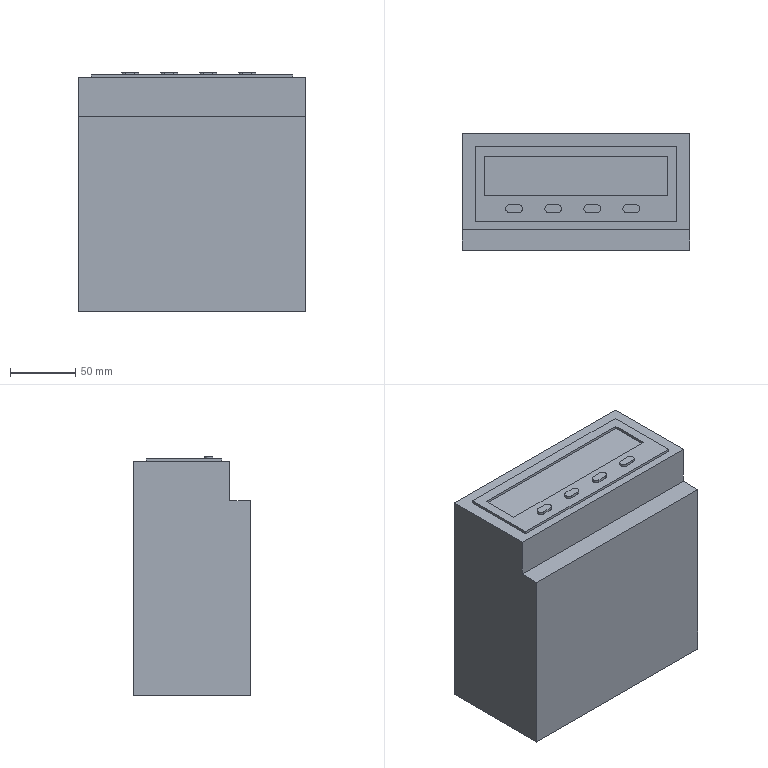Component | SolidWorks | Chassis-2 | 1 solid | 38 faces | box 175 x 90 x 184 mm | volume 2760814 mm3 | plane 30 | cylinder 8 | commonest cylinder face diameters 6 x8
build123d program:
from build123d import *

# Parameters (mm, degrees)
SKETCH1_W           = 175
SKETCH1_H           = 150
BOSS_EXTRUDE1_DEPTH = 90
SKETCH2_W           = 175
SKETCH2_H           = 73.952
BOSS_EXTRUDE2_DEPTH = 30
SKETCH3_W           = 155
SKETCH3_H           = 57.955
SKETCH3_W_2         = 141
SKETCH3_H_2         = 30
BOSS_EXTRUDE3_DEPTH = 2
BOSS_EXTRUDE4_DEPTH = 2


with BuildPart() as part:
    # Sketch1 → Boss-Extrude1 (new body)
    with BuildSketch(Plane.XY):
        with Locations((-127.5, 15)):
            Rectangle(SKETCH1_W, SKETCH1_H)
    extrude(amount=BOSS_EXTRUDE1_DEPTH)

    # Sketch2 → Boss-Extrude2 (add)
    with BuildSketch(Plane.XZ.offset(60)):
        with Locations((-127.5, 53.024)):
            Rectangle(SKETCH2_W, SKETCH2_H)
    extrude(amount=BOSS_EXTRUDE2_DEPTH)

    # Sketch3 → Boss-Extrude3 (add)
    with BuildSketch(Plane.XZ.offset(90)):
        with Locations((-127.5, 51.026)):
            Rectangle(SKETCH3_W, SKETCH3_H)
        with Locations((-127.5, 57.048)):
            Rectangle(SKETCH3_W_2, SKETCH3_H_2, mode=Mode.SUBTRACT)
    extrude(amount=BOSS_EXTRUDE3_DEPTH)

    # Sketch4 → Boss-Extrude4 (add)
    with BuildSketch(Plane.XZ.offset(92)):
        with BuildLine():
            Line((-178.5, 35.048), (-171.5, 35.048))
            ThreePointArc((-171.5, 35.048), (-168.5, 32.048), (-171.5, 29.048))
            Line((-171.5, 29.048), (-178.5, 29.048))
            ThreePointArc((-178.5, 29.048), (-181.5, 32.048), (-178.5, 35.048))
        make_face()
        with BuildLine():
            Line((-148.5, 35.048), (-141.5, 35.048))
            ThreePointArc((-141.5, 35.048), (-138.5, 32.048), (-141.5, 29.048))
            Line((-141.5, 29.048), (-148.5, 29.048))
            ThreePointArc((-148.5, 29.048), (-151.5, 32.048), (-148.5, 35.048))
        make_face()
        with BuildLine():
            Line((-118.5, 35.048), (-111.5, 35.048))
            ThreePointArc((-111.5, 35.048), (-108.5, 32.048), (-111.5, 29.048))
            Line((-111.5, 29.048), (-118.5, 29.048))
            ThreePointArc((-118.5, 29.048), (-121.5, 32.048), (-118.5, 35.048))
        make_face()
        with BuildLine():
            Line((-88.5, 35.048), (-81.5, 35.048))
            ThreePointArc((-81.5, 35.048), (-78.5, 32.048), (-81.5, 29.048))
            Line((-81.5, 29.048), (-88.5, 29.048))
            ThreePointArc((-88.5, 29.048), (-91.5, 32.048), (-88.5, 35.048))
        make_face()
    extrude(amount=BOSS_EXTRUDE4_DEPTH)


solid = part.part

# Placed as in the assembly
solid = solid.moved(Location((-695, 260, -10), (-90, 0, 0)))
STEP:
#1=COLOUR_RGB('',0.7922,0.8196,0.9333);
#2=FILL_AREA_STYLE_COLOUR('',#1);
#3=FILL_AREA_STYLE('',(#2));
#4=SURFACE_STYLE_FILL_AREA(#3);
#5=SURFACE_SIDE_STYLE('',(#4));
#6=SURFACE_STYLE_USAGE(.BOTH.,#5);
#7=PRESENTATION_STYLE_ASSIGNMENT((#6));
#8=CARTESIAN_POINT('',(-35.433,11.104,3.228));
#9=VERTEX_POINT('',#8);
#10=CARTESIAN_POINT('',(-29.331,11.104,3.228));
#11=VERTEX_POINT('',#10);
#12=CARTESIAN_POINT('',(-35.433,11.104,3.228));
#13=DIRECTION('',(1.,0.,0.));
#14=VECTOR('',#13,39.37);
#15=LINE('',#12,#14);
#16=EDGE_CURVE('',#9,#11,#15,.T.);
#17=ORIENTED_EDGE('',*,*,#16,.T.);
#18=CARTESIAN_POINT('',(-29.331,13.386,3.228));
#19=VERTEX_POINT('',#18);
#20=CARTESIAN_POINT('',(-29.331,11.104,3.228));
#21=DIRECTION('',(-0.,1.,0.));
#22=VECTOR('',#21,39.37);
#23=LINE('',#20,#22);
#24=EDGE_CURVE('',#11,#19,#23,.T.);
#25=ORIENTED_EDGE('',*,*,#24,.T.);
#26=CARTESIAN_POINT('',(-35.433,13.386,3.228));
#27=VERTEX_POINT('',#26);
#28=CARTESIAN_POINT('',(-29.331,13.386,3.228));
#29=DIRECTION('',(-1.,-0.,0.));
#30=VECTOR('',#29,39.37);
#31=LINE('',#28,#30);
#32=EDGE_CURVE('',#19,#27,#31,.T.);
#33=ORIENTED_EDGE('',*,*,#32,.T.);
#34=CARTESIAN_POINT('',(-35.433,13.386,3.228));
#35=DIRECTION('',(0.,-1.,0.));
#36=VECTOR('',#35,39.37);
#37=LINE('',#34,#36);
#38=EDGE_CURVE('',#27,#9,#37,.T.);
#39=ORIENTED_EDGE('',*,*,#38,.T.);
#40=EDGE_LOOP('',(#17,#25,#33,#39));
#41=FACE_OUTER_BOUND('',#40,.T.);
#42=CARTESIAN_POINT('',(-29.606,13.073,3.228));
#43=VERTEX_POINT('',#42);
#44=CARTESIAN_POINT('',(-35.157,13.073,3.228));
#45=VERTEX_POINT('',#44);
#46=CARTESIAN_POINT('',(-29.606,13.073,3.228));
#47=DIRECTION('',(-1.,-0.,0.));
#48=VECTOR('',#47,39.37);
#49=LINE('',#46,#48);
#50=EDGE_CURVE('',#43,#45,#49,.T.);
#51=ORIENTED_EDGE('',*,*,#50,.F.);
#52=CARTESIAN_POINT('',(-29.606,11.892,3.228));
#53=VERTEX_POINT('',#52);
#54=CARTESIAN_POINT('',(-29.606,13.073,3.228));
#55=DIRECTION('',(-0.,1.,0.));
#56=VECTOR('',#55,39.37);
#57=LINE('',#54,#56);
#58=EDGE_CURVE('',#53,#43,#57,.T.);
#59=ORIENTED_EDGE('',*,*,#58,.F.);
#60=CARTESIAN_POINT('',(-35.157,11.892,3.228));
#61=VERTEX_POINT('',#60);
#62=CARTESIAN_POINT('',(-29.606,11.892,3.228));
#63=DIRECTION('',(1.,0.,0.));
#64=VECTOR('',#63,39.37);
#65=LINE('',#62,#64);
#66=EDGE_CURVE('',#61,#53,#65,.T.);
#67=ORIENTED_EDGE('',*,*,#66,.F.);
#68=CARTESIAN_POINT('',(-35.157,13.073,3.228));
#69=DIRECTION('',(0.,-1.,0.));
#70=VECTOR('',#69,39.37);
#71=LINE('',#68,#70);
#72=EDGE_CURVE('',#45,#61,#71,.T.);
#73=ORIENTED_EDGE('',*,*,#72,.F.);
#74=EDGE_LOOP('',(#51,#59,#67,#73));
#75=FACE_BOUND('',#74,.T.);
#76=CARTESIAN_POINT('',(-34.39,11.38,3.228));
#77=VERTEX_POINT('',#76);
#78=CARTESIAN_POINT('',(-34.114,11.38,3.228));
#79=VERTEX_POINT('',#78);
#80=CARTESIAN_POINT('',(-34.39,11.38,3.228));
#81=DIRECTION('',(1.,0.,0.));
#82=VECTOR('',#81,39.37);
#83=LINE('',#80,#82);
#84=EDGE_CURVE('',#77,#79,#83,.T.);
#85=ORIENTED_EDGE('',*,*,#84,.F.);
#86=CARTESIAN_POINT('',(-34.39,11.616,3.228));
#87=VERTEX_POINT('',#86);
#88=CARTESIAN_POINT('',(-34.39,11.498,3.228));
#89=DIRECTION('',(0.,0.,1.));
#90=DIRECTION('',(0.,-1.,0.));
#91=AXIS2_PLACEMENT_3D('',#88,#89,#90);
#92=CIRCLE('',#91,0.1181);
#93=EDGE_CURVE('',#87,#77,#92,.T.);
#94=ORIENTED_EDGE('',*,*,#93,.F.);
#95=CARTESIAN_POINT('',(-34.114,11.616,3.228));
#96=VERTEX_POINT('',#95);
#97=CARTESIAN_POINT('',(-34.39,11.616,3.228));
#98=DIRECTION('',(-1.,-0.,0.));
#99=VECTOR('',#98,39.37);
#100=LINE('',#97,#99);
#101=EDGE_CURVE('',#96,#87,#100,.T.);
#102=ORIENTED_EDGE('',*,*,#101,.F.);
#103=CARTESIAN_POINT('',(-34.114,11.498,3.228));
#104=DIRECTION('',(0.,0.,1.));
#105=DIRECTION('',(0.,-1.,0.));
#106=AXIS2_PLACEMENT_3D('',#103,#104,#105);
#107=CIRCLE('',#106,0.1181);
#108=EDGE_CURVE('',#79,#96,#107,.T.);
#109=ORIENTED_EDGE('',*,*,#108,.F.);
#110=EDGE_LOOP('',(#85,#94,#102,#109));
#111=FACE_BOUND('',#110,.T.);
#112=CARTESIAN_POINT('',(-33.209,11.38,3.228));
#113=VERTEX_POINT('',#112);
#114=CARTESIAN_POINT('',(-32.933,11.38,3.228));
#115=VERTEX_POINT('',#114);
#116=CARTESIAN_POINT('',(-33.209,11.38,3.228));
#117=DIRECTION('',(1.,0.,0.));
#118=VECTOR('',#117,39.37);
#119=LINE('',#116,#118);
#120=EDGE_CURVE('',#113,#115,#119,.T.);
#121=ORIENTED_EDGE('',*,*,#120,.F.);
#122=CARTESIAN_POINT('',(-33.209,11.616,3.228));
#123=VERTEX_POINT('',#122);
#124=CARTESIAN_POINT('',(-33.209,11.498,3.228));
#125=DIRECTION('',(0.,0.,1.));
#126=DIRECTION('',(0.,-1.,0.));
#127=AXIS2_PLACEMENT_3D('',#124,#125,#126);
#128=CIRCLE('',#127,0.1181);
#129=EDGE_CURVE('',#123,#113,#128,.T.);
#130=ORIENTED_EDGE('',*,*,#129,.F.);
#131=CARTESIAN_POINT('',(-32.933,11.616,3.228));
#132=VERTEX_POINT('',#131);
#133=CARTESIAN_POINT('',(-33.209,11.616,3.228));
#134=DIRECTION('',(-1.,-0.,0.));
#135=VECTOR('',#134,39.37);
#136=LINE('',#133,#135);
#137=EDGE_CURVE('',#132,#123,#136,.T.);
#138=ORIENTED_EDGE('',*,*,#137,.F.);
#139=CARTESIAN_POINT('',(-32.933,11.498,3.228));
#140=DIRECTION('',(0.,0.,1.));
#141=DIRECTION('',(0.,-1.,0.));
#142=AXIS2_PLACEMENT_3D('',#139,#140,#141);
#143=CIRCLE('',#142,0.1181);
#144=EDGE_CURVE('',#115,#132,#143,.T.);
#145=ORIENTED_EDGE('',*,*,#144,.F.);
#146=EDGE_LOOP('',(#121,#130,#138,#145));
#147=FACE_BOUND('',#146,.T.);
#148=CARTESIAN_POINT('',(-32.028,11.38,3.228));
#149=VERTEX_POINT('',#148);
#150=CARTESIAN_POINT('',(-31.752,11.38,3.228));
#151=VERTEX_POINT('',#150);
#152=CARTESIAN_POINT('',(-32.028,11.38,3.228));
#153=DIRECTION('',(1.,0.,0.));
#154=VECTOR('',#153,39.37);
#155=LINE('',#152,#154);
#156=EDGE_CURVE('',#149,#151,#155,.T.);
#157=ORIENTED_EDGE('',*,*,#156,.F.);
#158=CARTESIAN_POINT('',(-32.028,11.616,3.228));
#159=VERTEX_POINT('',#158);
#160=CARTESIAN_POINT('',(-32.028,11.498,3.228));
#161=DIRECTION('',(0.,0.,1.));
#162=DIRECTION('',(0.,-1.,0.));
#163=AXIS2_PLACEMENT_3D('',#160,#161,#162);
#164=CIRCLE('',#163,0.1181);
#165=EDGE_CURVE('',#159,#149,#164,.T.);
#166=ORIENTED_EDGE('',*,*,#165,.F.);
#167=CARTESIAN_POINT('',(-31.752,11.616,3.228));
#168=VERTEX_POINT('',#167);
#169=CARTESIAN_POINT('',(-32.028,11.616,3.228));
#170=DIRECTION('',(-1.,-0.,0.));
#171=VECTOR('',#170,39.37);
#172=LINE('',#169,#171);
#173=EDGE_CURVE('',#168,#159,#172,.T.);
#174=ORIENTED_EDGE('',*,*,#173,.F.);
#175=CARTESIAN_POINT('',(-31.752,11.498,3.228));
#176=DIRECTION('',(0.,0.,1.));
#177=DIRECTION('',(0.,-1.,0.));
#178=AXIS2_PLACEMENT_3D('',#175,#176,#177);
#179=CIRCLE('',#178,0.1181);
#180=EDGE_CURVE('',#151,#168,#179,.T.);
#181=ORIENTED_EDGE('',*,*,#180,.F.);
#182=EDGE_LOOP('',(#157,#166,#174,#181));
#183=FACE_BOUND('',#182,.T.);
#184=CARTESIAN_POINT('',(-30.846,11.38,3.228));
#185=VERTEX_POINT('',#184);
#186=CARTESIAN_POINT('',(-30.571,11.38,3.228));
#187=VERTEX_POINT('',#186);
#188=CARTESIAN_POINT('',(-30.846,11.38,3.228));
#189=DIRECTION('',(1.,0.,0.));
#190=VECTOR('',#189,39.37);
#191=LINE('',#188,#190);
#192=EDGE_CURVE('',#185,#187,#191,.T.);
#193=ORIENTED_EDGE('',*,*,#192,.F.);
#194=CARTESIAN_POINT('',(-30.846,11.616,3.228));
#195=VERTEX_POINT('',#194);
#196=CARTESIAN_POINT('',(-30.846,11.498,3.228));
#197=DIRECTION('',(0.,0.,1.));
#198=DIRECTION('',(0.,-1.,0.));
#199=AXIS2_PLACEMENT_3D('',#196,#197,#198);
#200=CIRCLE('',#199,0.1181);
#201=EDGE_CURVE('',#195,#185,#200,.T.);
#202=ORIENTED_EDGE('',*,*,#201,.F.);
#203=CARTESIAN_POINT('',(-30.571,11.616,3.228));
#204=VERTEX_POINT('',#203);
#205=CARTESIAN_POINT('',(-30.846,11.616,3.228));
#206=DIRECTION('',(-1.,-0.,0.));
#207=VECTOR('',#206,39.37);
#208=LINE('',#205,#207);
#209=EDGE_CURVE('',#204,#195,#208,.T.);
#210=ORIENTED_EDGE('',*,*,#209,.F.);
#211=CARTESIAN_POINT('',(-30.571,11.498,3.228));
#212=DIRECTION('',(0.,0.,1.));
#213=DIRECTION('',(0.,-1.,0.));
#214=AXIS2_PLACEMENT_3D('',#211,#212,#213);
#215=CIRCLE('',#214,0.1181);
#216=EDGE_CURVE('',#187,#204,#215,.T.);
#217=ORIENTED_EDGE('',*,*,#216,.F.);
#218=EDGE_LOOP('',(#193,#202,#210,#217));
#219=FACE_BOUND('',#218,.T.);
#220=CARTESIAN_POINT('',(-27.362,10.236,3.228));
#221=DIRECTION('',(0.,0.,1.));
#222=DIRECTION('',(0.,-1.,0.));
#223=AXIS2_PLACEMENT_3D('',#220,#221,#222);
#224=PLANE('',#223);
#225=ADVANCED_FACE('',(#41,#75,#111,#147,#183,#219),#224,.T.);
#226=CARTESIAN_POINT('',(-28.937,10.868,3.15));
#227=VERTEX_POINT('',#226);
#228=CARTESIAN_POINT('',(-28.937,13.78,3.15));
#229=VERTEX_POINT('',#228);
#230=CARTESIAN_POINT('',(-28.937,13.78,3.15));
#231=DIRECTION('',(-0.,1.,0.));
#232=VECTOR('',#231,39.37);
#233=LINE('',#230,#232);
#234=EDGE_CURVE('',#227,#229,#233,.T.);
#235=ORIENTED_EDGE('',*,*,#234,.T.);
#236=CARTESIAN_POINT('',(-35.827,13.78,3.15));
#237=VERTEX_POINT('',#236);
#238=CARTESIAN_POINT('',(-28.937,13.78,3.15));
#239=DIRECTION('',(-1.,-0.,0.));
#240=VECTOR('',#239,39.37);
#241=LINE('',#238,#240);
#242=EDGE_CURVE('',#229,#237,#241,.T.);
#243=ORIENTED_EDGE('',*,*,#242,.T.);
#244=CARTESIAN_POINT('',(-35.827,10.868,3.15));
#245=VERTEX_POINT('',#244);
#246=CARTESIAN_POINT('',(-35.827,13.78,3.15));
#247=DIRECTION('',(-0.,-1.,0.));
#248=VECTOR('',#247,39.37);
#249=LINE('',#246,#248);
#250=EDGE_CURVE('',#237,#245,#249,.T.);
#251=ORIENTED_EDGE('',*,*,#250,.T.);
#252=CARTESIAN_POINT('',(-28.937,10.868,3.15));
#253=DIRECTION('',(1.,0.,0.));
#254=VECTOR('',#253,39.37);
#255=LINE('',#252,#254);
#256=EDGE_CURVE('',#245,#227,#255,.T.);
#257=ORIENTED_EDGE('',*,*,#256,.T.);
#258=EDGE_LOOP('',(#235,#243,#251,#257));
#259=FACE_OUTER_BOUND('',#258,.T.);
#260=CARTESIAN_POINT('',(-35.433,11.104,3.15));
#261=VERTEX_POINT('',#260);
#262=CARTESIAN_POINT('',(-29.331,11.104,3.15));
#263=VERTEX_POINT('',#262);
#264=CARTESIAN_POINT('',(-35.433,11.104,3.15));
#265=DIRECTION('',(1.,0.,0.));
#266=VECTOR('',#265,39.37);
#267=LINE('',#264,#266);
#268=EDGE_CURVE('',#261,#263,#267,.T.);
#269=ORIENTED_EDGE('',*,*,#268,.F.);
#270=CARTESIAN_POINT('',(-35.433,13.386,3.15));
#271=VERTEX_POINT('',#270);
#272=CARTESIAN_POINT('',(-35.433,13.386,3.15));
#273=DIRECTION('',(0.,-1.,0.));
#274=VECTOR('',#273,39.37);
#275=LINE('',#272,#274);
#276=EDGE_CURVE('',#271,#261,#275,.T.);
#277=ORIENTED_EDGE('',*,*,#276,.F.);
#278=CARTESIAN_POINT('',(-29.331,13.386,3.15));
#279=VERTEX_POINT('',#278);
#280=CARTESIAN_POINT('',(-29.331,13.386,3.15));
#281=DIRECTION('',(-1.,-0.,0.));
#282=VECTOR('',#281,39.37);
#283=LINE('',#280,#282);
#284=EDGE_CURVE('',#279,#271,#283,.T.);
#285=ORIENTED_EDGE('',*,*,#284,.F.);
#286=CARTESIAN_POINT('',(-29.331,11.104,3.15));
#287=DIRECTION('',(-0.,1.,0.));
#288=VECTOR('',#287,39.37);
#289=LINE('',#286,#288);
#290=EDGE_CURVE('',#263,#279,#289,.T.);
#291=ORIENTED_EDGE('',*,*,#290,.F.);
#292=EDGE_LOOP('',(#269,#277,#285,#291));
#293=FACE_BOUND('',#292,.T.);
#294=CARTESIAN_POINT('',(-27.362,10.236,3.15));
#295=DIRECTION('',(0.,0.,-1.));
#296=DIRECTION('',(-0.,1.,0.));
#297=AXIS2_PLACEMENT_3D('',#294,#295,#296);
#298=PLANE('',#297);
#299=ADVANCED_FACE('',(#259,#293),#298,.F.);
#300=CARTESIAN_POINT('',(-35.827,10.868,1.969));
#301=VERTEX_POINT('',#300);
#302=CARTESIAN_POINT('',(-28.937,10.868,1.969));
#303=VERTEX_POINT('',#302);
#304=CARTESIAN_POINT('',(-28.937,10.868,1.969));
#305=DIRECTION('',(1.,0.,0.));
#306=VECTOR('',#305,39.37);
#307=LINE('',#304,#306);
#308=EDGE_CURVE('',#301,#303,#307,.T.);
#309=ORIENTED_EDGE('',*,*,#308,.F.);
#310=CARTESIAN_POINT('',(-35.827,10.236,1.969));
#311=VERTEX_POINT('',#310);
#312=CARTESIAN_POINT('',(-35.827,13.78,1.969));
#313=DIRECTION('',(0.,-1.,0.));
#314=VECTOR('',#313,39.37);
#315=LINE('',#312,#314);
#316=EDGE_CURVE('',#301,#311,#315,.T.);
#317=ORIENTED_EDGE('',*,*,#316,.T.);
#318=CARTESIAN_POINT('',(-28.937,10.236,1.969));
#319=VERTEX_POINT('',#318);
#320=CARTESIAN_POINT('',(-35.827,10.236,1.969));
#321=DIRECTION('',(1.,0.,-0.));
#322=VECTOR('',#321,39.37);
#323=LINE('',#320,#322);
#324=EDGE_CURVE('',#311,#319,#323,.T.);
#325=ORIENTED_EDGE('',*,*,#324,.T.);
#326=CARTESIAN_POINT('',(-28.937,13.78,1.969));
#327=DIRECTION('',(0.,-1.,0.));
#328=VECTOR('',#327,39.37);
#329=LINE('',#326,#328);
#330=EDGE_CURVE('',#303,#319,#329,.T.);
#331=ORIENTED_EDGE('',*,*,#330,.F.);
#332=EDGE_LOOP('',(#309,#317,#325,#331));
#333=FACE_OUTER_BOUND('',#332,.T.);
#334=CARTESIAN_POINT('',(-35.827,13.78,1.969));
#335=DIRECTION('',(-0.,-0.,-1.));
#336=DIRECTION('',(-1.,-0.,0.));
#337=AXIS2_PLACEMENT_3D('',#334,#335,#336);
#338=PLANE('',#337);
#339=ADVANCED_FACE('',(#333),#338,.F.);
#340=CARTESIAN_POINT('',(-35.827,10.236,-3.937));
#341=VERTEX_POINT('',#340);
#342=CARTESIAN_POINT('',(-35.827,10.236,-3.937));
#343=DIRECTION('',(0.,0.,1.));
#344=VECTOR('',#343,39.37);
#345=LINE('',#342,#344);
#346=EDGE_CURVE('',#341,#311,#345,.T.);
#347=ORIENTED_EDGE('',*,*,#346,.T.);
#348=ORIENTED_EDGE('',*,*,#316,.F.);
#349=CARTESIAN_POINT('',(-35.827,10.868,3.15));
#350=DIRECTION('',(0.,0.,-1.));
#351=VECTOR('',#350,39.37);
#352=LINE('',#349,#351);
#353=EDGE_CURVE('',#245,#301,#352,.T.);
#354=ORIENTED_EDGE('',*,*,#353,.F.);
#355=ORIENTED_EDGE('',*,*,#250,.F.);
#356=CARTESIAN_POINT('',(-35.827,13.78,-3.937));
#357=VERTEX_POINT('',#356);
#358=CARTESIAN_POINT('',(-35.827,13.78,-3.937));
#359=DIRECTION('',(0.,0.,1.));
#360=VECTOR('',#359,39.37);
#361=LINE('',#358,#360);
#362=EDGE_CURVE('',#357,#237,#361,.T.);
#363=ORIENTED_EDGE('',*,*,#362,.F.);
#364=CARTESIAN_POINT('',(-35.827,13.78,-3.937));
#365=DIRECTION('',(0.,-1.,0.));
#366=VECTOR('',#365,39.37);
#367=LINE('',#364,#366);
#368=EDGE_CURVE('',#357,#341,#367,.T.);
#369=ORIENTED_EDGE('',*,*,#368,.T.);
#370=EDGE_LOOP('',(#347,#348,#354,#355,#363,#369));
#371=FACE_OUTER_BOUND('',#370,.T.);
#372=CARTESIAN_POINT('',(-35.827,13.78,-3.937));
#373=DIRECTION('',(1.,0.,-0.));
#374=DIRECTION('',(-0.,-0.,-1.));
#375=AXIS2_PLACEMENT_3D('',#372,#373,#374);
#376=PLANE('',#375);
#377=ADVANCED_FACE('',(#371),#376,.F.);
#378=CARTESIAN_POINT('',(-28.937,10.236,-3.937));
#379=VERTEX_POINT('',#378);
#380=CARTESIAN_POINT('',(-28.937,10.236,-3.937));
#381=DIRECTION('',(-0.,-0.,-1.));
#382=VECTOR('',#381,39.37);
#383=LINE('',#380,#382);
#384=EDGE_CURVE('',#319,#379,#383,.T.);
#385=ORIENTED_EDGE('',*,*,#384,.T.);
#386=CARTESIAN_POINT('',(-28.937,13.78,-3.937));
#387=VERTEX_POINT('',#386);
#388=CARTESIAN_POINT('',(-28.937,13.78,-3.937));
#389=DIRECTION('',(0.,-1.,0.));
#390=VECTOR('',#389,39.37);
#391=LINE('',#388,#390);
#392=EDGE_CURVE('',#387,#379,#391,.T.);
#393=ORIENTED_EDGE('',*,*,#392,.F.);
#394=CARTESIAN_POINT('',(-28.937,13.78,-3.937));
#395=DIRECTION('',(-0.,-0.,-1.));
#396=VECTOR('',#395,39.37);
#397=LINE('',#394,#396);
#398=EDGE_CURVE('',#229,#387,#397,.T.);
#399=ORIENTED_EDGE('',*,*,#398,.F.);
#400=ORIENTED_EDGE('',*,*,#234,.F.);
#401=CARTESIAN_POINT('',(-28.937,10.868,3.15));
#402=DIRECTION('',(0.,0.,-1.));
#403=VECTOR('',#402,39.37);
#404=LINE('',#401,#403);
#405=EDGE_CURVE('',#227,#303,#404,.T.);
#406=ORIENTED_EDGE('',*,*,#405,.T.);
#407=ORIENTED_EDGE('',*,*,#330,.T.);
#408=EDGE_LOOP('',(#385,#393,#399,#400,#406,#407));
#409=FACE_OUTER_BOUND('',#408,.T.);
#410=CARTESIAN_POINT('',(-28.937,13.78,-3.937));
#411=DIRECTION('',(-1.,-0.,0.));
#412=DIRECTION('',(0.,0.,1.));
#413=AXIS2_PLACEMENT_3D('',#410,#411,#412);
#414=PLANE('',#413);
#415=ADVANCED_FACE('',(#409),#414,.F.);
#416=CARTESIAN_POINT('',(-35.827,10.236,-3.937));
#417=DIRECTION('',(-1.,-0.,0.));
#418=VECTOR('',#417,39.37);
#419=LINE('',#416,#418);
#420=EDGE_CURVE('',#379,#341,#419,.T.);
#421=ORIENTED_EDGE('',*,*,#420,.T.);
#422=ORIENTED_EDGE('',*,*,#368,.F.);
#423=CARTESIAN_POINT('',(-35.827,13.78,-3.937));
#424=DIRECTION('',(-1.,-0.,0.));
#425=VECTOR('',#424,39.37);
#426=LINE('',#423,#425);
#427=EDGE_CURVE('',#387,#357,#426,.T.);
#428=ORIENTED_EDGE('',*,*,#427,.F.);
#429=ORIENTED_EDGE('',*,*,#392,.T.);
#430=EDGE_LOOP('',(#421,#422,#428,#429));
#431=FACE_OUTER_BOUND('',#430,.T.);
#432=CARTESIAN_POINT('',(-35.827,13.78,-3.937));
#433=DIRECTION('',(0.,0.,1.));
#434=DIRECTION('',(0.,-1.,0.));
#435=AXIS2_PLACEMENT_3D('',#432,#433,#434);
#436=PLANE('',#435);
#437=ADVANCED_FACE('',(#431),#436,.F.);
#438=ORIENTED_EDGE('',*,*,#362,.T.);
#439=ORIENTED_EDGE('',*,*,#242,.F.);
#440=ORIENTED_EDGE('',*,*,#398,.T.);
#441=ORIENTED_EDGE('',*,*,#427,.T.);
#442=EDGE_LOOP('',(#438,#439,#440,#441));
#443=FACE_OUTER_BOUND('',#442,.T.);
#444=CARTESIAN_POINT('',(-27.362,13.78,-0.3937));
#445=DIRECTION('',(-0.,1.,0.));
#446=DIRECTION('',(1.,0.,0.));
#447=AXIS2_PLACEMENT_3D('',#444,#445,#446);
#448=PLANE('',#447);
#449=ADVANCED_FACE('',(#443),#448,.T.);
#450=ORIENTED_EDGE('',*,*,#346,.F.);
#451=ORIENTED_EDGE('',*,*,#420,.F.);
#452=ORIENTED_EDGE('',*,*,#384,.F.);
#453=ORIENTED_EDGE('',*,*,#324,.F.);
#454=EDGE_LOOP('',(#450,#451,#452,#453));
#455=FACE_OUTER_BOUND('',#454,.T.);
#456=CARTESIAN_POINT('',(-27.362,10.236,-0.3937));
#457=DIRECTION('',(-0.,1.,0.));
#458=DIRECTION('',(1.,0.,0.));
#459=AXIS2_PLACEMENT_3D('',#456,#457,#458);
#460=PLANE('',#459);
#461=ADVANCED_FACE('',(#455),#460,.F.);
#462=ORIENTED_EDGE('',*,*,#308,.T.);
#463=ORIENTED_EDGE('',*,*,#405,.F.);
#464=ORIENTED_EDGE('',*,*,#256,.F.);
#465=ORIENTED_EDGE('',*,*,#353,.T.);
#466=EDGE_LOOP('',(#462,#463,#464,#465));
#467=FACE_OUTER_BOUND('',#466,.T.);
#468=CARTESIAN_POINT('',(-28.937,10.868,3.15));
#469=DIRECTION('',(-0.,1.,0.));
#470=DIRECTION('',(1.,0.,0.));
#471=AXIS2_PLACEMENT_3D('',#468,#469,#470);
#472=PLANE('',#471);
#473=ADVANCED_FACE('',(#467),#472,.F.);
#474=ORIENTED_EDGE('',*,*,#268,.T.);
#475=CARTESIAN_POINT('',(-29.331,11.104,3.228));
#476=DIRECTION('',(0.,0.,-1.));
#477=VECTOR('',#476,39.37);
#478=LINE('',#475,#477);
#479=EDGE_CURVE('',#11,#263,#478,.T.);
#480=ORIENTED_EDGE('',*,*,#479,.F.);
#481=ORIENTED_EDGE('',*,*,#16,.F.);
#482=CARTESIAN_POINT('',(-35.433,11.104,3.228));
#483=DIRECTION('',(0.,0.,-1.));
#484=VECTOR('',#483,39.37);
#485=LINE('',#482,#484);
#486=EDGE_CURVE('',#9,#261,#485,.T.);
#487=ORIENTED_EDGE('',*,*,#486,.T.);
#488=EDGE_LOOP('',(#474,#480,#481,#487));
#489=FACE_OUTER_BOUND('',#488,.T.);
#490=CARTESIAN_POINT('',(-35.433,11.104,3.228));
#491=DIRECTION('',(-0.,1.,0.));
#492=DIRECTION('',(1.,0.,0.));
#493=AXIS2_PLACEMENT_3D('',#490,#491,#492);
#494=PLANE('',#493);
#495=ADVANCED_FACE('',(#489),#494,.F.);
#496=ORIENTED_EDGE('',*,*,#290,.T.);
#497=CARTESIAN_POINT('',(-29.331,13.386,3.228));
#498=DIRECTION('',(0.,0.,-1.));
#499=VECTOR('',#498,39.37);
#500=LINE('',#497,#499);
#501=EDGE_CURVE('',#19,#279,#500,.T.);
#502=ORIENTED_EDGE('',*,*,#501,.F.);
#503=ORIENTED_EDGE('',*,*,#24,.F.);
#504=ORIENTED_EDGE('',*,*,#479,.T.);
#505=EDGE_LOOP('',(#496,#502,#503,#504));
#506=FACE_OUTER_BOUND('',#505,.T.);
#507=CARTESIAN_POINT('',(-29.331,11.104,3.228));
#508=DIRECTION('',(-1.,-0.,0.));
#509=DIRECTION('',(-0.,1.,0.));
#510=AXIS2_PLACEMENT_3D('',#507,#508,#509);
#511=PLANE('',#510);
#512=ADVANCED_FACE('',(#506),#511,.F.);
#513=ORIENTED_EDGE('',*,*,#284,.T.);
#514=CARTESIAN_POINT('',(-35.433,13.386,3.228));
#515=DIRECTION('',(0.,0.,-1.));
#516=VECTOR('',#515,39.37);
#517=LINE('',#514,#516);
#518=EDGE_CURVE('',#27,#271,#517,.T.);
#519=ORIENTED_EDGE('',*,*,#518,.F.);
#520=ORIENTED_EDGE('',*,*,#32,.F.);
#521=ORIENTED_EDGE('',*,*,#501,.T.);
#522=EDGE_LOOP('',(#513,#519,#520,#521));
#523=FACE_OUTER_BOUND('',#522,.T.);
#524=CARTESIAN_POINT('',(-29.331,13.386,3.228));
#525=DIRECTION('',(0.,-1.,0.));
#526=DIRECTION('',(-1.,-0.,0.));
#527=AXIS2_PLACEMENT_3D('',#524,#525,#526);
#528=PLANE('',#527);
#529=ADVANCED_FACE('',(#523),#528,.F.);
#530=ORIENTED_EDGE('',*,*,#276,.T.);
#531=ORIENTED_EDGE('',*,*,#486,.F.);
#532=ORIENTED_EDGE('',*,*,#38,.F.);
#533=ORIENTED_EDGE('',*,*,#518,.T.);
#534=EDGE_LOOP('',(#530,#531,#532,#533));
#535=FACE_OUTER_BOUND('',#534,.T.);
#536=CARTESIAN_POINT('',(-35.433,13.386,3.228));
#537=DIRECTION('',(1.,0.,0.));
#538=DIRECTION('',(0.,-1.,0.));
#539=AXIS2_PLACEMENT_3D('',#536,#537,#538);
#540=PLANE('',#539);
#541=ADVANCED_FACE('',(#535),#540,.F.);
#542=CARTESIAN_POINT('',(-29.606,11.892,3.15));
#543=VERTEX_POINT('',#542);
#544=CARTESIAN_POINT('',(-29.606,13.073,3.15));
#545=VERTEX_POINT('',#544);
#546=CARTESIAN_POINT('',(-29.606,13.073,3.15));
#547=DIRECTION('',(-0.,1.,0.));
#548=VECTOR('',#547,39.37);
#549=LINE('',#546,#548);
#550=EDGE_CURVE('',#543,#545,#549,.T.);
#551=ORIENTED_EDGE('',*,*,#550,.F.);
#552=CARTESIAN_POINT('',(-29.606,11.892,3.228));
#553=DIRECTION('',(0.,0.,-1.));
#554=VECTOR('',#553,39.37);
#555=LINE('',#552,#554);
#556=EDGE_CURVE('',#53,#543,#555,.T.);
#557=ORIENTED_EDGE('',*,*,#556,.F.);
#558=ORIENTED_EDGE('',*,*,#58,.T.);
#559=CARTESIAN_POINT('',(-29.606,13.073,3.228));
#560=DIRECTION('',(0.,0.,-1.));
#561=VECTOR('',#560,39.37);
#562=LINE('',#559,#561);
#563=EDGE_CURVE('',#43,#545,#562,.T.);
#564=ORIENTED_EDGE('',*,*,#563,.T.);
#565=EDGE_LOOP('',(#551,#557,#558,#564));
#566=FACE_OUTER_BOUND('',#565,.T.);
#567=CARTESIAN_POINT('',(-29.606,13.073,3.228));
#568=DIRECTION('',(-1.,-0.,0.));
#569=DIRECTION('',(-0.,1.,0.));
#570=AXIS2_PLACEMENT_3D('',#567,#568,#569);
#571=PLANE('',#570);
#572=ADVANCED_FACE('',(#566),#571,.T.);
#573=CARTESIAN_POINT('',(-35.157,13.073,3.15));
#574=VERTEX_POINT('',#573);
#575=CARTESIAN_POINT('',(-29.606,13.073,3.15));
#576=DIRECTION('',(-1.,-0.,0.));
#577=VECTOR('',#576,39.37);
#578=LINE('',#575,#577);
#579=EDGE_CURVE('',#545,#574,#578,.T.);
#580=ORIENTED_EDGE('',*,*,#579,.F.);
#581=ORIENTED_EDGE('',*,*,#563,.F.);
#582=ORIENTED_EDGE('',*,*,#50,.T.);
#583=CARTESIAN_POINT('',(-35.157,13.073,3.228));
#584=DIRECTION('',(0.,0.,-1.));
#585=VECTOR('',#584,39.37);
#586=LINE('',#583,#585);
#587=EDGE_CURVE('',#45,#574,#586,.T.);
#588=ORIENTED_EDGE('',*,*,#587,.T.);
#589=EDGE_LOOP('',(#580,#581,#582,#588));
#590=FACE_OUTER_BOUND('',#589,.T.);
#591=CARTESIAN_POINT('',(-29.606,13.073,3.228));
#592=DIRECTION('',(0.,-1.,0.));
#593=DIRECTION('',(-1.,-0.,0.));
#594=AXIS2_PLACEMENT_3D('',#591,#592,#593);
#595=PLANE('',#594);
#596=ADVANCED_FACE('',(#590),#595,.T.);
#597=CARTESIAN_POINT('',(-35.157,11.892,3.15));
#598=VERTEX_POINT('',#597);
#599=CARTESIAN_POINT('',(-35.157,13.073,3.15));
#600=DIRECTION('',(0.,-1.,0.));
#601=VECTOR('',#600,39.37);
#602=LINE('',#599,#601);
#603=EDGE_CURVE('',#574,#598,#602,.T.);
#604=ORIENTED_EDGE('',*,*,#603,.F.);
#605=ORIENTED_EDGE('',*,*,#587,.F.);
#606=ORIENTED_EDGE('',*,*,#72,.T.);
#607=CARTESIAN_POINT('',(-35.157,11.892,3.228));
#608=DIRECTION('',(0.,0.,-1.));
#609=VECTOR('',#608,39.37);
#610=LINE('',#607,#609);
#611=EDGE_CURVE('',#61,#598,#610,.T.);
#612=ORIENTED_EDGE('',*,*,#611,.T.);
#613=EDGE_LOOP('',(#604,#605,#606,#612));
#614=FACE_OUTER_BOUND('',#613,.T.);
#615=CARTESIAN_POINT('',(-35.157,13.073,3.228));
#616=DIRECTION('',(1.,0.,0.));
#617=DIRECTION('',(0.,-1.,0.));
#618=AXIS2_PLACEMENT_3D('',#615,#616,#617);
#619=PLANE('',#618);
#620=ADVANCED_FACE('',(#614),#619,.T.);
#621=CARTESIAN_POINT('',(-29.606,11.892,3.15));
#622=DIRECTION('',(1.,0.,0.));
#623=VECTOR('',#622,39.37);
#624=LINE('',#621,#623);
#625=EDGE_CURVE('',#598,#543,#624,.T.);
#626=ORIENTED_EDGE('',*,*,#625,.F.);
#627=ORIENTED_EDGE('',*,*,#611,.F.);
#628=ORIENTED_EDGE('',*,*,#66,.T.);
#629=ORIENTED_EDGE('',*,*,#556,.T.);
#630=EDGE_LOOP('',(#626,#627,#628,#629));
#631=FACE_OUTER_BOUND('',#630,.T.);
#632=CARTESIAN_POINT('',(-29.606,11.892,3.228));
#633=DIRECTION('',(-0.,1.,0.));
#634=DIRECTION('',(1.,0.,0.));
#635=AXIS2_PLACEMENT_3D('',#632,#633,#634);
#636=PLANE('',#635);
#637=ADVANCED_FACE('',(#631),#636,.T.);
#638=ORIENTED_EDGE('',*,*,#625,.T.);
#639=ORIENTED_EDGE('',*,*,#550,.T.);
#640=ORIENTED_EDGE('',*,*,#579,.T.);
#641=ORIENTED_EDGE('',*,*,#603,.T.);
#642=EDGE_LOOP('',(#638,#639,#640,#641));
#643=FACE_OUTER_BOUND('',#642,.T.);
#644=CARTESIAN_POINT('',(-27.362,10.236,3.15));
#645=DIRECTION('',(0.,0.,-1.));
#646=DIRECTION('',(-0.,1.,0.));
#647=AXIS2_PLACEMENT_3D('',#644,#645,#646);
#648=PLANE('',#647);
#649=ADVANCED_FACE('',(#643),#648,.F.);
#650=ORIENTED_EDGE('',*,*,#93,.T.);
#651=CARTESIAN_POINT('',(-34.39,11.38,3.307));
#652=VERTEX_POINT('',#651);
#653=CARTESIAN_POINT('',(-34.39,11.38,3.307));
#654=DIRECTION('',(0.,0.,-1.));
#655=VECTOR('',#654,39.37);
#656=LINE('',#653,#655);
#657=EDGE_CURVE('',#652,#77,#656,.T.);
#658=ORIENTED_EDGE('',*,*,#657,.F.);
#659=CARTESIAN_POINT('',(-34.39,11.616,3.307));
#660=VERTEX_POINT('',#659);
#661=CARTESIAN_POINT('',(-34.39,11.498,3.307));
#662=DIRECTION('',(0.,0.,1.));
#663=DIRECTION('',(0.,-1.,0.));
#664=AXIS2_PLACEMENT_3D('',#661,#662,#663);
#665=CIRCLE('',#664,0.1181);
#666=EDGE_CURVE('',#660,#652,#665,.T.);
#667=ORIENTED_EDGE('',*,*,#666,.F.);
#668=CARTESIAN_POINT('',(-34.39,11.616,3.307));
#669=DIRECTION('',(0.,0.,-1.));
#670=VECTOR('',#669,39.37);
#671=LINE('',#668,#670);
#672=EDGE_CURVE('',#660,#87,#671,.T.);
#673=ORIENTED_EDGE('',*,*,#672,.T.);
#674=EDGE_LOOP('',(#650,#658,#667,#673));
#675=FACE_OUTER_BOUND('',#674,.T.);
#676=CARTESIAN_POINT('',(-34.39,11.498,3.307));
#677=DIRECTION('',(0.,0.,-1.));
#678=DIRECTION('',(0.,1.,0.));
#679=AXIS2_PLACEMENT_3D('',#676,#677,#678);
#680=CYLINDRICAL_SURFACE('',#679,0.1181);
#681=ADVANCED_FACE('',(#675),#680,.T.);
#682=ORIENTED_EDGE('',*,*,#84,.T.);
#683=CARTESIAN_POINT('',(-34.114,11.38,3.307));
#684=VERTEX_POINT('',#683);
#685=CARTESIAN_POINT('',(-34.114,11.38,3.307));
#686=DIRECTION('',(0.,0.,-1.));
#687=VECTOR('',#686,39.37);
#688=LINE('',#685,#687);
#689=EDGE_CURVE('',#684,#79,#688,.T.);
#690=ORIENTED_EDGE('',*,*,#689,.F.);
#691=CARTESIAN_POINT('',(-34.39,11.38,3.307));
#692=DIRECTION('',(1.,0.,0.));
#693=VECTOR('',#692,39.37);
#694=LINE('',#691,#693);
#695=EDGE_CURVE('',#652,#684,#694,.T.);
#696=ORIENTED_EDGE('',*,*,#695,.F.);
#697=ORIENTED_EDGE('',*,*,#657,.T.);
#698=EDGE_LOOP('',(#682,#690,#696,#697));
#699=FACE_OUTER_BOUND('',#698,.T.);
#700=CARTESIAN_POINT('',(-34.39,11.38,3.307));
#701=DIRECTION('',(-0.,1.,0.));
#702=DIRECTION('',(1.,0.,0.));
#703=AXIS2_PLACEMENT_3D('',#700,#701,#702);
#704=PLANE('',#703);
#705=ADVANCED_FACE('',(#699),#704,.F.);
#706=ORIENTED_EDGE('',*,*,#108,.T.);
#707=CARTESIAN_POINT('',(-34.114,11.616,3.307));
#708=VERTEX_POINT('',#707);
#709=CARTESIAN_POINT('',(-34.114,11.616,3.307));
#710=DIRECTION('',(0.,0.,-1.));
#711=VECTOR('',#710,39.37);
#712=LINE('',#709,#711);
#713=EDGE_CURVE('',#708,#96,#712,.T.);
#714=ORIENTED_EDGE('',*,*,#713,.F.);
#715=CARTESIAN_POINT('',(-34.114,11.498,3.307));
#716=DIRECTION('',(0.,0.,1.));
#717=DIRECTION('',(0.,-1.,0.));
#718=AXIS2_PLACEMENT_3D('',#715,#716,#717);
#719=CIRCLE('',#718,0.1181);
#720=EDGE_CURVE('',#684,#708,#719,.T.);
#721=ORIENTED_EDGE('',*,*,#720,.F.);
#722=ORIENTED_EDGE('',*,*,#689,.T.);
#723=EDGE_LOOP('',(#706,#714,#721,#722));
#724=FACE_OUTER_BOUND('',#723,.T.);
#725=CARTESIAN_POINT('',(-34.114,11.498,3.307));
#726=DIRECTION('',(0.,0.,-1.));
#727=DIRECTION('',(0.,1.,0.));
#728=AXIS2_PLACEMENT_3D('',#725,#726,#727);
#729=CYLINDRICAL_SURFACE('',#728,0.1181);
#730=ADVANCED_FACE('',(#724),#729,.T.);
#731=ORIENTED_EDGE('',*,*,#101,.T.);
#732=ORIENTED_EDGE('',*,*,#672,.F.);
#733=CARTESIAN_POINT('',(-34.39,11.616,3.307));
#734=DIRECTION('',(-1.,-0.,0.));
#735=VECTOR('',#734,39.37);
#736=LINE('',#733,#735);
#737=EDGE_CURVE('',#708,#660,#736,.T.);
#738=ORIENTED_EDGE('',*,*,#737,.F.);
#739=ORIENTED_EDGE('',*,*,#713,.T.);
#740=EDGE_LOOP('',(#731,#732,#738,#739));
#741=FACE_OUTER_BOUND('',#740,.T.);
#742=CARTESIAN_POINT('',(-34.39,11.616,3.307));
#743=DIRECTION('',(0.,-1.,0.));
#744=DIRECTION('',(-1.,-0.,0.));
#745=AXIS2_PLACEMENT_3D('',#742,#743,#744);
#746=PLANE('',#745);
#747=ADVANCED_FACE('',(#741),#746,.F.);
#748=ORIENTED_EDGE('',*,*,#666,.T.);
#749=ORIENTED_EDGE('',*,*,#695,.T.);
#750=ORIENTED_EDGE('',*,*,#720,.T.);
#751=ORIENTED_EDGE('',*,*,#737,.T.);
#752=EDGE_LOOP('',(#748,#749,#750,#751));
#753=FACE_OUTER_BOUND('',#752,.T.);
#754=CARTESIAN_POINT('',(-34.39,11.498,3.307));
#755=DIRECTION('',(0.,0.,1.));
#756=DIRECTION('',(0.,-1.,0.));
#757=AXIS2_PLACEMENT_3D('',#754,#755,#756);
#758=PLANE('',#757);
#759=ADVANCED_FACE('',(#753),#758,.T.);
#760=ORIENTED_EDGE('',*,*,#129,.T.);
#761=CARTESIAN_POINT('',(-33.209,11.38,3.307));
#762=VERTEX_POINT('',#761);
#763=CARTESIAN_POINT('',(-33.209,11.38,3.307));
#764=DIRECTION('',(0.,0.,-1.));
#765=VECTOR('',#764,39.37);
#766=LINE('',#763,#765);
#767=EDGE_CURVE('',#762,#113,#766,.T.);
#768=ORIENTED_EDGE('',*,*,#767,.F.);
#769=CARTESIAN_POINT('',(-33.209,11.616,3.307));
#770=VERTEX_POINT('',#769);
#771=CARTESIAN_POINT('',(-33.209,11.498,3.307));
#772=DIRECTION('',(0.,0.,1.));
#773=DIRECTION('',(0.,-1.,0.));
#774=AXIS2_PLACEMENT_3D('',#771,#772,#773);
#775=CIRCLE('',#774,0.1181);
#776=EDGE_CURVE('',#770,#762,#775,.T.);
#777=ORIENTED_EDGE('',*,*,#776,.F.);
#778=CARTESIAN_POINT('',(-33.209,11.616,3.307));
#779=DIRECTION('',(0.,0.,-1.));
#780=VECTOR('',#779,39.37);
#781=LINE('',#778,#780);
#782=EDGE_CURVE('',#770,#123,#781,.T.);
#783=ORIENTED_EDGE('',*,*,#782,.T.);
#784=EDGE_LOOP('',(#760,#768,#777,#783));
#785=FACE_OUTER_BOUND('',#784,.T.);
#786=CARTESIAN_POINT('',(-33.209,11.498,3.307));
#787=DIRECTION('',(0.,0.,-1.));
#788=DIRECTION('',(0.,1.,0.));
#789=AXIS2_PLACEMENT_3D('',#786,#787,#788);
#790=CYLINDRICAL_SURFACE('',#789,0.1181);
#791=ADVANCED_FACE('',(#785),#790,.T.);
#792=ORIENTED_EDGE('',*,*,#120,.T.);
#793=CARTESIAN_POINT('',(-32.933,11.38,3.307));
#794=VERTEX_POINT('',#793);
#795=CARTESIAN_POINT('',(-32.933,11.38,3.307));
#796=DIRECTION('',(0.,0.,-1.));
#797=VECTOR('',#796,39.37);
#798=LINE('',#795,#797);
#799=EDGE_CURVE('',#794,#115,#798,.T.);
#800=ORIENTED_EDGE('',*,*,#799,.F.);
#801=CARTESIAN_POINT('',(-33.209,11.38,3.307));
#802=DIRECTION('',(1.,0.,0.));
#803=VECTOR('',#802,39.37);
#804=LINE('',#801,#803);
#805=EDGE_CURVE('',#762,#794,#804,.T.);
#806=ORIENTED_EDGE('',*,*,#805,.F.);
#807=ORIENTED_EDGE('',*,*,#767,.T.);
#808=EDGE_LOOP('',(#792,#800,#806,#807));
#809=FACE_OUTER_BOUND('',#808,.T.);
#810=CARTESIAN_POINT('',(-33.209,11.38,3.307));
#811=DIRECTION('',(-0.,1.,0.));
#812=DIRECTION('',(1.,0.,0.));
#813=AXIS2_PLACEMENT_3D('',#810,#811,#812);
#814=PLANE('',#813);
#815=ADVANCED_FACE('',(#809),#814,.F.);
#816=ORIENTED_EDGE('',*,*,#144,.T.);
#817=CARTESIAN_POINT('',(-32.933,11.616,3.307));
#818=VERTEX_POINT('',#817);
#819=CARTESIAN_POINT('',(-32.933,11.616,3.307));
#820=DIRECTION('',(0.,0.,-1.));
#821=VECTOR('',#820,39.37);
#822=LINE('',#819,#821);
#823=EDGE_CURVE('',#818,#132,#822,.T.);
#824=ORIENTED_EDGE('',*,*,#823,.F.);
#825=CARTESIAN_POINT('',(-32.933,11.498,3.307));
#826=DIRECTION('',(0.,0.,1.));
#827=DIRECTION('',(0.,-1.,0.));
#828=AXIS2_PLACEMENT_3D('',#825,#826,#827);
#829=CIRCLE('',#828,0.1181);
#830=EDGE_CURVE('',#794,#818,#829,.T.);
#831=ORIENTED_EDGE('',*,*,#830,.F.);
#832=ORIENTED_EDGE('',*,*,#799,.T.);
#833=EDGE_LOOP('',(#816,#824,#831,#832));
#834=FACE_OUTER_BOUND('',#833,.T.);
#835=CARTESIAN_POINT('',(-32.933,11.498,3.307));
#836=DIRECTION('',(0.,0.,-1.));
#837=DIRECTION('',(0.,1.,0.));
#838=AXIS2_PLACEMENT_3D('',#835,#836,#837);
#839=CYLINDRICAL_SURFACE('',#838,0.1181);
#840=ADVANCED_FACE('',(#834),#839,.T.);
#841=ORIENTED_EDGE('',*,*,#137,.T.);
#842=ORIENTED_EDGE('',*,*,#782,.F.);
#843=CARTESIAN_POINT('',(-33.209,11.616,3.307));
#844=DIRECTION('',(-1.,-0.,0.));
#845=VECTOR('',#844,39.37);
#846=LINE('',#843,#845);
#847=EDGE_CURVE('',#818,#770,#846,.T.);
#848=ORIENTED_EDGE('',*,*,#847,.F.);
#849=ORIENTED_EDGE('',*,*,#823,.T.);
#850=EDGE_LOOP('',(#841,#842,#848,#849));
#851=FACE_OUTER_BOUND('',#850,.T.);
#852=CARTESIAN_POINT('',(-33.209,11.616,3.307));
#853=DIRECTION('',(0.,-1.,0.));
#854=DIRECTION('',(-1.,-0.,0.));
#855=AXIS2_PLACEMENT_3D('',#852,#853,#854);
#856=PLANE('',#855);
#857=ADVANCED_FACE('',(#851),#856,.F.);
#858=ORIENTED_EDGE('',*,*,#776,.T.);
#859=ORIENTED_EDGE('',*,*,#805,.T.);
#860=ORIENTED_EDGE('',*,*,#830,.T.);
#861=ORIENTED_EDGE('',*,*,#847,.T.);
#862=EDGE_LOOP('',(#858,#859,#860,#861));
#863=FACE_OUTER_BOUND('',#862,.T.);
#864=CARTESIAN_POINT('',(-33.209,11.498,3.307));
#865=DIRECTION('',(0.,0.,1.));
#866=DIRECTION('',(0.,-1.,0.));
#867=AXIS2_PLACEMENT_3D('',#864,#865,#866);
#868=PLANE('',#867);
#869=ADVANCED_FACE('',(#863),#868,.T.);
#870=ORIENTED_EDGE('',*,*,#165,.T.);
#871=CARTESIAN_POINT('',(-32.028,11.38,3.307));
#872=VERTEX_POINT('',#871);
#873=CARTESIAN_POINT('',(-32.028,11.38,3.307));
#874=DIRECTION('',(0.,0.,-1.));
#875=VECTOR('',#874,39.37);
#876=LINE('',#873,#875);
#877=EDGE_CURVE('',#872,#149,#876,.T.);
#878=ORIENTED_EDGE('',*,*,#877,.F.);
#879=CARTESIAN_POINT('',(-32.028,11.616,3.307));
#880=VERTEX_POINT('',#879);
#881=CARTESIAN_POINT('',(-32.028,11.498,3.307));
#882=DIRECTION('',(0.,0.,1.));
#883=DIRECTION('',(0.,-1.,0.));
#884=AXIS2_PLACEMENT_3D('',#881,#882,#883);
#885=CIRCLE('',#884,0.1181);
#886=EDGE_CURVE('',#880,#872,#885,.T.);
#887=ORIENTED_EDGE('',*,*,#886,.F.);
#888=CARTESIAN_POINT('',(-32.028,11.616,3.307));
#889=DIRECTION('',(0.,0.,-1.));
#890=VECTOR('',#889,39.37);
#891=LINE('',#888,#890);
#892=EDGE_CURVE('',#880,#159,#891,.T.);
#893=ORIENTED_EDGE('',*,*,#892,.T.);
#894=EDGE_LOOP('',(#870,#878,#887,#893));
#895=FACE_OUTER_BOUND('',#894,.T.);
#896=CARTESIAN_POINT('',(-32.028,11.498,3.307));
#897=DIRECTION('',(0.,0.,-1.));
#898=DIRECTION('',(0.,1.,0.));
#899=AXIS2_PLACEMENT_3D('',#896,#897,#898);
#900=CYLINDRICAL_SURFACE('',#899,0.1181);
#901=ADVANCED_FACE('',(#895),#900,.T.);
#902=ORIENTED_EDGE('',*,*,#156,.T.);
#903=CARTESIAN_POINT('',(-31.752,11.38,3.307));
#904=VERTEX_POINT('',#903);
#905=CARTESIAN_POINT('',(-31.752,11.38,3.307));
#906=DIRECTION('',(0.,0.,-1.));
#907=VECTOR('',#906,39.37);
#908=LINE('',#905,#907);
#909=EDGE_CURVE('',#904,#151,#908,.T.);
#910=ORIENTED_EDGE('',*,*,#909,.F.);
#911=CARTESIAN_POINT('',(-32.028,11.38,3.307));
#912=DIRECTION('',(1.,0.,0.));
#913=VECTOR('',#912,39.37);
#914=LINE('',#911,#913);
#915=EDGE_CURVE('',#872,#904,#914,.T.);
#916=ORIENTED_EDGE('',*,*,#915,.F.);
#917=ORIENTED_EDGE('',*,*,#877,.T.);
#918=EDGE_LOOP('',(#902,#910,#916,#917));
#919=FACE_OUTER_BOUND('',#918,.T.);
#920=CARTESIAN_POINT('',(-32.028,11.38,3.307));
#921=DIRECTION('',(-0.,1.,0.));
#922=DIRECTION('',(1.,0.,0.));
#923=AXIS2_PLACEMENT_3D('',#920,#921,#922);
#924=PLANE('',#923);
#925=ADVANCED_FACE('',(#919),#924,.F.);
#926=ORIENTED_EDGE('',*,*,#180,.T.);
#927=CARTESIAN_POINT('',(-31.752,11.616,3.307));
#928=VERTEX_POINT('',#927);
#929=CARTESIAN_POINT('',(-31.752,11.616,3.307));
#930=DIRECTION('',(0.,0.,-1.));
#931=VECTOR('',#930,39.37);
#932=LINE('',#929,#931);
#933=EDGE_CURVE('',#928,#168,#932,.T.);
#934=ORIENTED_EDGE('',*,*,#933,.F.);
#935=CARTESIAN_POINT('',(-31.752,11.498,3.307));
#936=DIRECTION('',(0.,0.,1.));
#937=DIRECTION('',(0.,-1.,0.));
#938=AXIS2_PLACEMENT_3D('',#935,#936,#937);
#939=CIRCLE('',#938,0.1181);
#940=EDGE_CURVE('',#904,#928,#939,.T.);
#941=ORIENTED_EDGE('',*,*,#940,.F.);
#942=ORIENTED_EDGE('',*,*,#909,.T.);
#943=EDGE_LOOP('',(#926,#934,#941,#942));
#944=FACE_OUTER_BOUND('',#943,.T.);
#945=CARTESIAN_POINT('',(-31.752,11.498,3.307));
#946=DIRECTION('',(0.,0.,-1.));
#947=DIRECTION('',(0.,1.,0.));
#948=AXIS2_PLACEMENT_3D('',#945,#946,#947);
#949=CYLINDRICAL_SURFACE('',#948,0.1181);
#950=ADVANCED_FACE('',(#944),#949,.T.);
#951=ORIENTED_EDGE('',*,*,#173,.T.);
#952=ORIENTED_EDGE('',*,*,#892,.F.);
#953=CARTESIAN_POINT('',(-32.028,11.616,3.307));
#954=DIRECTION('',(-1.,-0.,0.));
#955=VECTOR('',#954,39.37);
#956=LINE('',#953,#955);
#957=EDGE_CURVE('',#928,#880,#956,.T.);
#958=ORIENTED_EDGE('',*,*,#957,.F.);
#959=ORIENTED_EDGE('',*,*,#933,.T.);
#960=EDGE_LOOP('',(#951,#952,#958,#959));
#961=FACE_OUTER_BOUND('',#960,.T.);
#962=CARTESIAN_POINT('',(-32.028,11.616,3.307));
#963=DIRECTION('',(0.,-1.,0.));
#964=DIRECTION('',(-1.,-0.,0.));
#965=AXIS2_PLACEMENT_3D('',#962,#963,#964);
#966=PLANE('',#965);
#967=ADVANCED_FACE('',(#961),#966,.F.);
#968=ORIENTED_EDGE('',*,*,#886,.T.);
#969=ORIENTED_EDGE('',*,*,#915,.T.);
#970=ORIENTED_EDGE('',*,*,#940,.T.);
#971=ORIENTED_EDGE('',*,*,#957,.T.);
#972=EDGE_LOOP('',(#968,#969,#970,#971));
#973=FACE_OUTER_BOUND('',#972,.T.);
#974=CARTESIAN_POINT('',(-32.028,11.498,3.307));
#975=DIRECTION('',(0.,0.,1.));
#976=DIRECTION('',(0.,-1.,0.));
#977=AXIS2_PLACEMENT_3D('',#974,#975,#976);
#978=PLANE('',#977);
#979=ADVANCED_FACE('',(#973),#978,.T.);
#980=ORIENTED_EDGE('',*,*,#201,.T.);
#981=CARTESIAN_POINT('',(-30.846,11.38,3.307));
#982=VERTEX_POINT('',#981);
#983=CARTESIAN_POINT('',(-30.846,11.38,3.307));
#984=DIRECTION('',(0.,0.,-1.));
#985=VECTOR('',#984,39.37);
#986=LINE('',#983,#985);
#987=EDGE_CURVE('',#982,#185,#986,.T.);
#988=ORIENTED_EDGE('',*,*,#987,.F.);
#989=CARTESIAN_POINT('',(-30.846,11.616,3.307));
#990=VERTEX_POINT('',#989);
#991=CARTESIAN_POINT('',(-30.846,11.498,3.307));
#992=DIRECTION('',(0.,0.,1.));
#993=DIRECTION('',(0.,-1.,0.));
#994=AXIS2_PLACEMENT_3D('',#991,#992,#993);
#995=CIRCLE('',#994,0.1181);
#996=EDGE_CURVE('',#990,#982,#995,.T.);
#997=ORIENTED_EDGE('',*,*,#996,.F.);
#998=CARTESIAN_POINT('',(-30.846,11.616,3.307));
#999=DIRECTION('',(0.,0.,-1.));
#1000=VECTOR('',#999,39.37);
#1001=LINE('',#998,#1000);
#1002=EDGE_CURVE('',#990,#195,#1001,.T.);
#1003=ORIENTED_EDGE('',*,*,#1002,.T.);
#1004=EDGE_LOOP('',(#980,#988,#997,#1003));
#1005=FACE_OUTER_BOUND('',#1004,.T.);
#1006=CARTESIAN_POINT('',(-30.846,11.498,3.307));
#1007=DIRECTION('',(0.,0.,-1.));
#1008=DIRECTION('',(0.,1.,0.));
#1009=AXIS2_PLACEMENT_3D('',#1006,#1007,#1008);
#1010=CYLINDRICAL_SURFACE('',#1009,0.1181);
#1011=ADVANCED_FACE('',(#1005),#1010,.T.);
#1012=ORIENTED_EDGE('',*,*,#192,.T.);
#1013=CARTESIAN_POINT('',(-30.571,11.38,3.307));
#1014=VERTEX_POINT('',#1013);
#1015=CARTESIAN_POINT('',(-30.571,11.38,3.307));
#1016=DIRECTION('',(0.,0.,-1.));
#1017=VECTOR('',#1016,39.37);
#1018=LINE('',#1015,#1017);
#1019=EDGE_CURVE('',#1014,#187,#1018,.T.);
#1020=ORIENTED_EDGE('',*,*,#1019,.F.);
#1021=CARTESIAN_POINT('',(-30.846,11.38,3.307));
#1022=DIRECTION('',(1.,0.,0.));
#1023=VECTOR('',#1022,39.37);
#1024=LINE('',#1021,#1023);
#1025=EDGE_CURVE('',#982,#1014,#1024,.T.);
#1026=ORIENTED_EDGE('',*,*,#1025,.F.);
#1027=ORIENTED_EDGE('',*,*,#987,.T.);
#1028=EDGE_LOOP('',(#1012,#1020,#1026,#1027));
#1029=FACE_OUTER_BOUND('',#1028,.T.);
#1030=CARTESIAN_POINT('',(-30.846,11.38,3.307));
#1031=DIRECTION('',(-0.,1.,0.));
#1032=DIRECTION('',(1.,0.,0.));
#1033=AXIS2_PLACEMENT_3D('',#1030,#1031,#1032);
#1034=PLANE('',#1033);
#1035=ADVANCED_FACE('',(#1029),#1034,.F.);
#1036=ORIENTED_EDGE('',*,*,#216,.T.);
#1037=CARTESIAN_POINT('',(-30.571,11.616,3.307));
#1038=VERTEX_POINT('',#1037);
#1039=CARTESIAN_POINT('',(-30.571,11.616,3.307));
#1040=DIRECTION('',(0.,0.,-1.));
#1041=VECTOR('',#1040,39.37);
#1042=LINE('',#1039,#1041);
#1043=EDGE_CURVE('',#1038,#204,#1042,.T.);
#1044=ORIENTED_EDGE('',*,*,#1043,.F.);
#1045=CARTESIAN_POINT('',(-30.571,11.498,3.307));
#1046=DIRECTION('',(0.,0.,1.));
#1047=DIRECTION('',(0.,-1.,0.));
#1048=AXIS2_PLACEMENT_3D('',#1045,#1046,#1047);
#1049=CIRCLE('',#1048,0.1181);
#1050=EDGE_CURVE('',#1014,#1038,#1049,.T.);
#1051=ORIENTED_EDGE('',*,*,#1050,.F.);
#1052=ORIENTED_EDGE('',*,*,#1019,.T.);
#1053=EDGE_LOOP('',(#1036,#1044,#1051,#1052));
#1054=FACE_OUTER_BOUND('',#1053,.T.);
#1055=CARTESIAN_POINT('',(-30.571,11.498,3.307));
#1056=DIRECTION('',(0.,0.,-1.));
#1057=DIRECTION('',(0.,1.,0.));
#1058=AXIS2_PLACEMENT_3D('',#1055,#1056,#1057);
#1059=CYLINDRICAL_SURFACE('',#1058,0.1181);
#1060=ADVANCED_FACE('',(#1054),#1059,.T.);
#1061=ORIENTED_EDGE('',*,*,#209,.T.);
#1062=ORIENTED_EDGE('',*,*,#1002,.F.);
#1063=CARTESIAN_POINT('',(-30.846,11.616,3.307));
#1064=DIRECTION('',(-1.,-0.,0.));
#1065=VECTOR('',#1064,39.37);
#1066=LINE('',#1063,#1065);
#1067=EDGE_CURVE('',#1038,#990,#1066,.T.);
#1068=ORIENTED_EDGE('',*,*,#1067,.F.);
#1069=ORIENTED_EDGE('',*,*,#1043,.T.);
#1070=EDGE_LOOP('',(#1061,#1062,#1068,#1069));
#1071=FACE_OUTER_BOUND('',#1070,.T.);
#1072=CARTESIAN_POINT('',(-30.846,11.616,3.307));
#1073=DIRECTION('',(0.,-1.,0.));
#1074=DIRECTION('',(-1.,-0.,0.));
#1075=AXIS2_PLACEMENT_3D('',#1072,#1073,#1074);
#1076=PLANE('',#1075);
#1077=ADVANCED_FACE('',(#1071),#1076,.F.);
#1078=ORIENTED_EDGE('',*,*,#996,.T.);
#1079=ORIENTED_EDGE('',*,*,#1025,.T.);
#1080=ORIENTED_EDGE('',*,*,#1050,.T.);
#1081=ORIENTED_EDGE('',*,*,#1067,.T.);
#1082=EDGE_LOOP('',(#1078,#1079,#1080,#1081));
#1083=FACE_OUTER_BOUND('',#1082,.T.);
#1084=CARTESIAN_POINT('',(-30.846,11.498,3.307));
#1085=DIRECTION('',(0.,0.,1.));
#1086=DIRECTION('',(0.,-1.,0.));
#1087=AXIS2_PLACEMENT_3D('',#1084,#1085,#1086);
#1088=PLANE('',#1087);
#1089=ADVANCED_FACE('',(#1083),#1088,.T.);
#1090=CLOSED_SHELL('',(#225,#299,#339,#377,#415,#437,#449,#461,#473,#495,#512,#529,#541,#572,#596,#620,#637,#649,#681,#705,#730,#747,#759,#791,#815,#840,#857,#869,#901,#925,#950,#967,#979,#1011,#1035,#1060,#1077,#1089));
#1091=MANIFOLD_SOLID_BREP('',#1090);
#1092=STYLED_ITEM('',(#7),#1091);
#1093=(LENGTH_UNIT()NAMED_UNIT(*)SI_UNIT($,.METRE.));
#1094=LENGTH_MEASURE_WITH_UNIT(LENGTH_MEASURE(0.0254),#1093);
#1095=DIMENSIONAL_EXPONENTS(1.,0.,0.,0.,0.,0.,0.);
#1096=(CONVERSION_BASED_UNIT('',#1094)LENGTH_UNIT()NAMED_UNIT(#1095));
#1097=UNCERTAINTY_MEASURE_WITH_UNIT(LENGTH_MEASURE(0.00001),#1096,'','');
#1098=(NAMED_UNIT(*)PLANE_ANGLE_UNIT()SI_UNIT($,.RADIAN.));
#1099=(NAMED_UNIT(*)SI_UNIT($,.STERADIAN.)SOLID_ANGLE_UNIT());
#1100=(GEOMETRIC_REPRESENTATION_CONTEXT(3)GLOBAL_UNCERTAINTY_ASSIGNED_CONTEXT((#1097))GLOBAL_UNIT_ASSIGNED_CONTEXT((#1096,#1098,#1099))REPRESENTATION_CONTEXT('',''));
#1101=MECHANICAL_DESIGN_GEOMETRIC_PRESENTATION_REPRESENTATION('',(#1092),#1100);
#1102=CARTESIAN_POINT('',(0.,0.,0.));
#1103=DIRECTION('',(0.,0.,1.));
#1104=DIRECTION('',(1.,0.,0.));
#1105=AXIS2_PLACEMENT_3D('',#1102,#1103,#1104);
#1106=(LENGTH_UNIT()NAMED_UNIT(*)SI_UNIT($,.METRE.));
#1107=LENGTH_MEASURE_WITH_UNIT(LENGTH_MEASURE(0.0254),#1106);
#1108=DIMENSIONAL_EXPONENTS(1.,0.,0.,0.,0.,0.,0.);
#1109=(CONVERSION_BASED_UNIT('',#1107)LENGTH_UNIT()NAMED_UNIT(#1108));
#1110=UNCERTAINTY_MEASURE_WITH_UNIT(LENGTH_MEASURE(0.00001),#1109,'','');
#1111=(NAMED_UNIT(*)PLANE_ANGLE_UNIT()SI_UNIT($,.RADIAN.));
#1112=(NAMED_UNIT(*)SI_UNIT($,.STERADIAN.)SOLID_ANGLE_UNIT());
#1113=(GEOMETRIC_REPRESENTATION_CONTEXT(3)GLOBAL_UNCERTAINTY_ASSIGNED_CONTEXT((#1110))GLOBAL_UNIT_ASSIGNED_CONTEXT((#1109,#1111,#1112))REPRESENTATION_CONTEXT('',''));
#1114=ADVANCED_BREP_SHAPE_REPRESENTATION('',(#1091,#1105),#1113);
#1115=PRESENTATION_LAYER_ASSIGNMENT('','',(#1092));